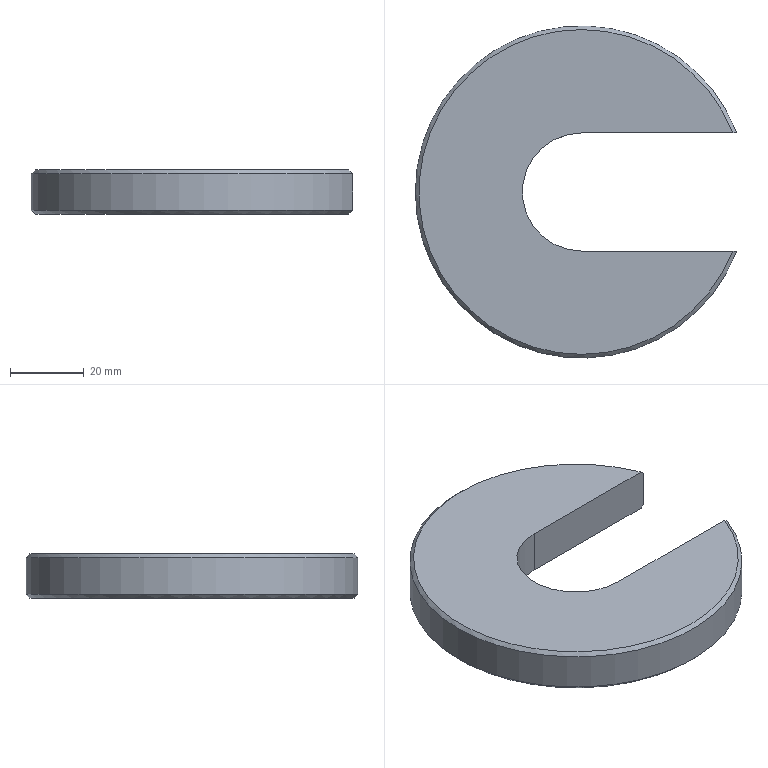Component | NX | QUICK_CHANGE_WASHER | 1 solid | 8 faces | box 87.06 x 90 x 12 mm | volume 54359 mm3 | plane 4 | cylinder 2 | cone 2 | commonest cylinder face diameters 32 x1 90 x1
STEP:
#1=CARTESIAN_POINT('',(0.,0.,0.));
#2=DIRECTION('',(0.,0.,1.));
#3=DIRECTION('',(1.,0.,0.));
#4=AXIS2_PLACEMENT_3D('',#1,#2,#3);
#5=CARTESIAN_POINT('',(42.059,-16.,129.));
#6=VERTEX_POINT('',#5);
#7=CARTESIAN_POINT('',(42.059,-16.,119.));
#8=VERTEX_POINT('',#7);
#9=CARTESIAN_POINT('',(42.059,-16.,130.));
#10=DIRECTION('',(0.,0.,-1.));
#11=VECTOR('',#10,1.);
#12=LINE('',#9,#11);
#13=CARTESIAN_POINT('',(42.059,-16.,130.));
#14=DIRECTION('',(0.,-1.,0.));
#15=DIRECTION('',(1.,0.,0.));
#16=AXIS2_PLACEMENT_3D('',#13,#14,#15);
#17=PLANE('',#16);
#18=CARTESIAN_POINT('',(0.,0.));
#19=DIRECTION('',(0.,-1.));
#20=VECTOR('',#19,1.);
#21=LINE('',#18,#20);
#22=(GEOMETRIC_REPRESENTATION_CONTEXT(2)PARAMETRIC_REPRESENTATION_CONTEXT()REPRESENTATION_CONTEXT('',''));
#23=DEFINITIONAL_REPRESENTATION('',(#21),#22);
#24=PCURVE('',#17,#23);
#25=CARTESIAN_POINT('',(-0.,0.,130.));
#26=DIRECTION('',(0.,0.,-1.));
#27=DIRECTION('',(0.,-1.,0.));
#28=AXIS2_PLACEMENT_3D('',#25,#26,#27);
#29=CYLINDRICAL_SURFACE('',#28,45.);
#30=CARTESIAN_POINT('',(-1.207,0.));
#31=DIRECTION('',(0.,1.));
#32=VECTOR('',#31,1.);
#33=LINE('',#30,#32);
#34=(GEOMETRIC_REPRESENTATION_CONTEXT(2)PARAMETRIC_REPRESENTATION_CONTEXT()REPRESENTATION_CONTEXT('',''));
#35=DEFINITIONAL_REPRESENTATION('',(#33),#34);
#36=PCURVE('',#29,#35);
#37=SURFACE_CURVE('',#12,(#24,#36),.PCURVE_S1.);
#38=EDGE_CURVE('',#6,#8,#37,.T.);
#39=ORIENTED_EDGE('',*,*,#38,.T.);
#40=CARTESIAN_POINT('',(40.988,-16.,118.));
#41=VERTEX_POINT('',#40);
#42=CARTESIAN_POINT('',(42.059,-16.,119.));
#43=CARTESIAN_POINT('',(41.703,-16.,118.666));
#44=CARTESIAN_POINT('',(41.345,-16.,118.333));
#45=CARTESIAN_POINT('',(40.988,-16.,118.));
#46=B_SPLINE_CURVE_WITH_KNOTS('',3,(#42,#43,#44,#45),.UNSPECIFIED.,.F.,.F.,(4,4),(0.,1.),.PIECEWISE_BEZIER_KNOTS.);
#47=CARTESIAN_POINT('',(0.,-11.));
#48=CARTESIAN_POINT('',(-0.357,-11.334));
#49=CARTESIAN_POINT('',(-0.7142,-11.667));
#50=CARTESIAN_POINT('',(-1.072,-12.));
#51=B_SPLINE_CURVE_WITH_KNOTS('',3,(#47,#48,#49,#50),.UNSPECIFIED.,.F.,.F.,(4,4),(0.,1.),.PIECEWISE_BEZIER_KNOTS.);
#52=(GEOMETRIC_REPRESENTATION_CONTEXT(2)PARAMETRIC_REPRESENTATION_CONTEXT()REPRESENTATION_CONTEXT('',''));
#53=DEFINITIONAL_REPRESENTATION('',(#51),#52);
#54=PCURVE('',#17,#53);
#55=CARTESIAN_POINT('',(-0.,0.,119.));
#56=DIRECTION('',(0.,0.,1.));
#57=DIRECTION('',(0.,1.,0.));
#58=AXIS2_PLACEMENT_3D('',#55,#56,#57);
#59=CONICAL_SURFACE('',#58,45.,0.7854);
#60=CARTESIAN_POINT('',(4.349,0.));
#61=CARTESIAN_POINT('',(4.34,-1.));
#62=B_SPLINE_CURVE_WITH_KNOTS('',1,(#60,#61),.UNSPECIFIED.,.F.,.F.,(2,2),(0.,1.),.PIECEWISE_BEZIER_KNOTS.);
#63=(GEOMETRIC_REPRESENTATION_CONTEXT(2)PARAMETRIC_REPRESENTATION_CONTEXT()REPRESENTATION_CONTEXT('',''));
#64=DEFINITIONAL_REPRESENTATION('',(#62),#63);
#65=PCURVE('',#59,#64);
#66=SURFACE_CURVE('',#46,(#54,#65),.PCURVE_S1.);
#67=EDGE_CURVE('',#8,#41,#66,.T.);
#68=ORIENTED_EDGE('',*,*,#67,.T.);
#69=CARTESIAN_POINT('',(-0.,-16.,118.));
#70=VERTEX_POINT('',#69);
#71=CARTESIAN_POINT('',(42.059,-16.,118.));
#72=DIRECTION('',(-1.,-0.,0.));
#73=VECTOR('',#72,1.);
#74=LINE('',#71,#73);
#75=CARTESIAN_POINT('',(0.,-12.));
#76=DIRECTION('',(-1.,0.));
#77=VECTOR('',#76,1.);
#78=LINE('',#75,#77);
#79=(GEOMETRIC_REPRESENTATION_CONTEXT(2)PARAMETRIC_REPRESENTATION_CONTEXT()REPRESENTATION_CONTEXT('',''));
#80=DEFINITIONAL_REPRESENTATION('',(#78),#79);
#81=PCURVE('',#17,#80);
#82=CARTESIAN_POINT('',(-0.,0.,118.));
#83=DIRECTION('',(0.,0.,-1.));
#84=DIRECTION('',(0.,-1.,0.));
#85=AXIS2_PLACEMENT_3D('',#82,#83,#84);
#86=PLANE('',#85);
#87=CARTESIAN_POINT('',(16.,-42.059));
#88=DIRECTION('',(0.,1.));
#89=VECTOR('',#88,1.);
#90=LINE('',#87,#89);
#91=(GEOMETRIC_REPRESENTATION_CONTEXT(2)PARAMETRIC_REPRESENTATION_CONTEXT()REPRESENTATION_CONTEXT('',''));
#92=DEFINITIONAL_REPRESENTATION('',(#90),#91);
#93=PCURVE('',#86,#92);
#94=SURFACE_CURVE('',#74,(#81,#93),.PCURVE_S1.);
#95=EDGE_CURVE('',#41,#70,#94,.T.);
#96=ORIENTED_EDGE('',*,*,#95,.T.);
#97=CARTESIAN_POINT('',(-0.,-16.,130.));
#98=VERTEX_POINT('',#97);
#99=CARTESIAN_POINT('',(-0.,-16.,130.));
#100=DIRECTION('',(0.,0.,-1.));
#101=VECTOR('',#100,1.);
#102=LINE('',#99,#101);
#103=CARTESIAN_POINT('',(-42.059,0.));
#104=DIRECTION('',(0.,-1.));
#105=VECTOR('',#104,1.);
#106=LINE('',#103,#105);
#107=(GEOMETRIC_REPRESENTATION_CONTEXT(2)PARAMETRIC_REPRESENTATION_CONTEXT()REPRESENTATION_CONTEXT('',''));
#108=DEFINITIONAL_REPRESENTATION('',(#106),#107);
#109=PCURVE('',#17,#108);
#110=CARTESIAN_POINT('',(-0.,0.,130.));
#111=DIRECTION('',(0.,0.,-1.));
#112=DIRECTION('',(0.,-1.,0.));
#113=AXIS2_PLACEMENT_3D('',#110,#111,#112);
#114=CYLINDRICAL_SURFACE('',#113,16.);
#115=CARTESIAN_POINT('',(0.,0.));
#116=DIRECTION('',(0.,1.));
#117=VECTOR('',#116,1.);
#118=LINE('',#115,#117);
#119=(GEOMETRIC_REPRESENTATION_CONTEXT(2)PARAMETRIC_REPRESENTATION_CONTEXT()REPRESENTATION_CONTEXT('',''));
#120=DEFINITIONAL_REPRESENTATION('',(#118),#119);
#121=PCURVE('',#114,#120);
#122=SURFACE_CURVE('',#102,(#109,#121),.PCURVE_S1.);
#123=EDGE_CURVE('',#98,#70,#122,.T.);
#124=ORIENTED_EDGE('',*,*,#123,.F.);
#125=CARTESIAN_POINT('',(40.988,-16.,130.));
#126=VERTEX_POINT('',#125);
#127=CARTESIAN_POINT('',(42.059,-16.,130.));
#128=DIRECTION('',(-1.,-0.,0.));
#129=VECTOR('',#128,1.);
#130=LINE('',#127,#129);
#131=CARTESIAN_POINT('',(0.,0.));
#132=DIRECTION('',(-1.,0.));
#133=VECTOR('',#132,1.);
#134=LINE('',#131,#133);
#135=(GEOMETRIC_REPRESENTATION_CONTEXT(2)PARAMETRIC_REPRESENTATION_CONTEXT()REPRESENTATION_CONTEXT('',''));
#136=DEFINITIONAL_REPRESENTATION('',(#134),#135);
#137=PCURVE('',#17,#136);
#138=CARTESIAN_POINT('',(-0.,0.,130.));
#139=DIRECTION('',(0.,0.,-1.));
#140=DIRECTION('',(0.,-1.,0.));
#141=AXIS2_PLACEMENT_3D('',#138,#139,#140);
#142=PLANE('',#141);
#143=CARTESIAN_POINT('',(16.,-42.059));
#144=DIRECTION('',(0.,1.));
#145=VECTOR('',#144,1.);
#146=LINE('',#143,#145);
#147=(GEOMETRIC_REPRESENTATION_CONTEXT(2)PARAMETRIC_REPRESENTATION_CONTEXT()REPRESENTATION_CONTEXT('',''));
#148=DEFINITIONAL_REPRESENTATION('',(#146),#147);
#149=PCURVE('',#142,#148);
#150=SURFACE_CURVE('',#130,(#137,#149),.PCURVE_S1.);
#151=EDGE_CURVE('',#126,#98,#150,.T.);
#152=ORIENTED_EDGE('',*,*,#151,.F.);
#153=CARTESIAN_POINT('',(40.988,-16.,130.));
#154=CARTESIAN_POINT('',(41.345,-16.,129.667));
#155=CARTESIAN_POINT('',(41.703,-16.,129.334));
#156=CARTESIAN_POINT('',(42.059,-16.,129.));
#157=B_SPLINE_CURVE_WITH_KNOTS('',3,(#153,#154,#155,#156),.UNSPECIFIED.,.F.,.F.,(4,4),(0.,1.),.PIECEWISE_BEZIER_KNOTS.);
#158=CARTESIAN_POINT('',(-1.072,0.));
#159=CARTESIAN_POINT('',(-0.7142,-0.333));
#160=CARTESIAN_POINT('',(-0.357,-0.6664));
#161=CARTESIAN_POINT('',(0.,-1.));
#162=B_SPLINE_CURVE_WITH_KNOTS('',3,(#158,#159,#160,#161),.UNSPECIFIED.,.F.,.F.,(4,4),(0.,1.),.PIECEWISE_BEZIER_KNOTS.);
#163=(GEOMETRIC_REPRESENTATION_CONTEXT(2)PARAMETRIC_REPRESENTATION_CONTEXT()REPRESENTATION_CONTEXT('',''));
#164=DEFINITIONAL_REPRESENTATION('',(#162),#163);
#165=PCURVE('',#17,#164);
#166=CARTESIAN_POINT('',(-0.,0.,130.));
#167=DIRECTION('',(0.,0.,-1.));
#168=DIRECTION('',(0.,-1.,0.));
#169=AXIS2_PLACEMENT_3D('',#166,#167,#168);
#170=CONICAL_SURFACE('',#169,44.,0.7854);
#171=CARTESIAN_POINT('',(-1.199,0.));
#172=CARTESIAN_POINT('',(-1.207,1.));
#173=B_SPLINE_CURVE_WITH_KNOTS('',1,(#171,#172),.UNSPECIFIED.,.F.,.F.,(2,2),(0.,1.),.PIECEWISE_BEZIER_KNOTS.);
#174=(GEOMETRIC_REPRESENTATION_CONTEXT(2)PARAMETRIC_REPRESENTATION_CONTEXT()REPRESENTATION_CONTEXT('',''));
#175=DEFINITIONAL_REPRESENTATION('',(#173),#174);
#176=PCURVE('',#170,#175);
#177=SURFACE_CURVE('',#157,(#165,#176),.PCURVE_S1.);
#178=EDGE_CURVE('',#126,#6,#177,.T.);
#179=ORIENTED_EDGE('',*,*,#178,.T.);
#180=EDGE_LOOP('',(#39,#68,#96,#124,#152,#179));
#181=FACE_BOUND('',#180,.T.);
#182=ADVANCED_FACE('',(#181),#17,.F.);
#183=ORIENTED_EDGE('',*,*,#123,.F.);
#184=CARTESIAN_POINT('',(-0.,16.,130.));
#185=VERTEX_POINT('',#184);
#186=CARTESIAN_POINT('',(-0.,0.,130.));
#187=DIRECTION('',(0.,0.,-1.));
#188=DIRECTION('',(-0.,1.,0.));
#189=AXIS2_PLACEMENT_3D('',#186,#187,#188);
#190=CIRCLE('',#189,16.);
#191=CARTESIAN_POINT('',(-3.142,0.));
#192=DIRECTION('',(1.,0.));
#193=VECTOR('',#192,1.);
#194=LINE('',#191,#193);
#195=(GEOMETRIC_REPRESENTATION_CONTEXT(2)PARAMETRIC_REPRESENTATION_CONTEXT()REPRESENTATION_CONTEXT('',''));
#196=DEFINITIONAL_REPRESENTATION('',(#194),#195);
#197=PCURVE('',#114,#196);
#198=CARTESIAN_POINT('',(0.,0.));
#199=DIRECTION('',(-1.,0.));
#200=AXIS2_PLACEMENT_2D('',#198,#199);
#201=CIRCLE('',#200,16.);
#202=(GEOMETRIC_REPRESENTATION_CONTEXT(2)PARAMETRIC_REPRESENTATION_CONTEXT()REPRESENTATION_CONTEXT('',''));
#203=DEFINITIONAL_REPRESENTATION('',(#201),#202);
#204=PCURVE('',#142,#203);
#205=SURFACE_CURVE('',#190,(#197,#204),.PCURVE_S1.);
#206=EDGE_CURVE('',#98,#185,#205,.T.);
#207=ORIENTED_EDGE('',*,*,#206,.T.);
#208=CARTESIAN_POINT('',(-0.,16.,118.));
#209=VERTEX_POINT('',#208);
#210=CARTESIAN_POINT('',(-0.,16.,130.));
#211=DIRECTION('',(0.,0.,-1.));
#212=VECTOR('',#211,1.);
#213=LINE('',#210,#212);
#214=CARTESIAN_POINT('',(3.142,0.));
#215=DIRECTION('',(0.,1.));
#216=VECTOR('',#215,1.);
#217=LINE('',#214,#216);
#218=(GEOMETRIC_REPRESENTATION_CONTEXT(2)PARAMETRIC_REPRESENTATION_CONTEXT()REPRESENTATION_CONTEXT('',''));
#219=DEFINITIONAL_REPRESENTATION('',(#217),#218);
#220=PCURVE('',#114,#219);
#221=CARTESIAN_POINT('',(-0.,16.,130.));
#222=DIRECTION('',(-0.,1.,0.));
#223=DIRECTION('',(-1.,-0.,0.));
#224=AXIS2_PLACEMENT_3D('',#221,#222,#223);
#225=PLANE('',#224);
#226=CARTESIAN_POINT('',(0.,0.));
#227=DIRECTION('',(0.,-1.));
#228=VECTOR('',#227,1.);
#229=LINE('',#226,#228);
#230=(GEOMETRIC_REPRESENTATION_CONTEXT(2)PARAMETRIC_REPRESENTATION_CONTEXT()REPRESENTATION_CONTEXT('',''));
#231=DEFINITIONAL_REPRESENTATION('',(#229),#230);
#232=PCURVE('',#225,#231);
#233=SURFACE_CURVE('',#213,(#220,#232),.PCURVE_S1.);
#234=EDGE_CURVE('',#185,#209,#233,.T.);
#235=ORIENTED_EDGE('',*,*,#234,.T.);
#236=CARTESIAN_POINT('',(-0.,0.,118.));
#237=DIRECTION('',(0.,0.,-1.));
#238=DIRECTION('',(-0.,1.,0.));
#239=AXIS2_PLACEMENT_3D('',#236,#237,#238);
#240=CIRCLE('',#239,16.);
#241=CARTESIAN_POINT('',(-3.142,12.));
#242=DIRECTION('',(1.,0.));
#243=VECTOR('',#242,1.);
#244=LINE('',#241,#243);
#245=(GEOMETRIC_REPRESENTATION_CONTEXT(2)PARAMETRIC_REPRESENTATION_CONTEXT()REPRESENTATION_CONTEXT('',''));
#246=DEFINITIONAL_REPRESENTATION('',(#244),#245);
#247=PCURVE('',#114,#246);
#248=CARTESIAN_POINT('',(0.,0.));
#249=DIRECTION('',(-1.,0.));
#250=AXIS2_PLACEMENT_2D('',#248,#249);
#251=CIRCLE('',#250,16.);
#252=(GEOMETRIC_REPRESENTATION_CONTEXT(2)PARAMETRIC_REPRESENTATION_CONTEXT()REPRESENTATION_CONTEXT('',''));
#253=DEFINITIONAL_REPRESENTATION('',(#251),#252);
#254=PCURVE('',#86,#253);
#255=SURFACE_CURVE('',#240,(#247,#254),.PCURVE_S1.);
#256=EDGE_CURVE('',#70,#209,#255,.T.);
#257=ORIENTED_EDGE('',*,*,#256,.F.);
#258=EDGE_LOOP('',(#183,#207,#235,#257));
#259=FACE_BOUND('',#258,.F.);
#260=ADVANCED_FACE('',(#259),#114,.F.);
#261=CARTESIAN_POINT('',(40.988,16.,118.));
#262=VERTEX_POINT('',#261);
#263=CARTESIAN_POINT('',(-0.,16.,118.));
#264=DIRECTION('',(1.,0.,0.));
#265=VECTOR('',#264,1.);
#266=LINE('',#263,#265);
#267=CARTESIAN_POINT('',(0.,-12.));
#268=DIRECTION('',(-1.,0.));
#269=VECTOR('',#268,1.);
#270=LINE('',#267,#269);
#271=(GEOMETRIC_REPRESENTATION_CONTEXT(2)PARAMETRIC_REPRESENTATION_CONTEXT()REPRESENTATION_CONTEXT('',''));
#272=DEFINITIONAL_REPRESENTATION('',(#270),#271);
#273=PCURVE('',#225,#272);
#274=CARTESIAN_POINT('',(-16.,-0.));
#275=DIRECTION('',(-0.,-1.));
#276=VECTOR('',#275,1.);
#277=LINE('',#274,#276);
#278=(GEOMETRIC_REPRESENTATION_CONTEXT(2)PARAMETRIC_REPRESENTATION_CONTEXT()REPRESENTATION_CONTEXT('',''));
#279=DEFINITIONAL_REPRESENTATION('',(#277),#278);
#280=PCURVE('',#86,#279);
#281=SURFACE_CURVE('',#266,(#273,#280),.PCURVE_S1.);
#282=EDGE_CURVE('',#209,#262,#281,.T.);
#283=ORIENTED_EDGE('',*,*,#282,.T.);
#284=CARTESIAN_POINT('',(42.059,16.,119.));
#285=VERTEX_POINT('',#284);
#286=CARTESIAN_POINT('',(40.988,16.,118.));
#287=CARTESIAN_POINT('',(41.345,16.,118.333));
#288=CARTESIAN_POINT('',(41.703,16.,118.666));
#289=CARTESIAN_POINT('',(42.059,16.,119.));
#290=B_SPLINE_CURVE_WITH_KNOTS('',3,(#286,#287,#288,#289),.UNSPECIFIED.,.F.,.F.,(4,4),(0.,1.),.PIECEWISE_BEZIER_KNOTS.);
#291=CARTESIAN_POINT('',(-40.988,-12.));
#292=CARTESIAN_POINT('',(-41.345,-11.667));
#293=CARTESIAN_POINT('',(-41.703,-11.334));
#294=CARTESIAN_POINT('',(-42.059,-11.));
#295=B_SPLINE_CURVE_WITH_KNOTS('',3,(#291,#292,#293,#294),.UNSPECIFIED.,.F.,.F.,(4,4),(0.,1.),.PIECEWISE_BEZIER_KNOTS.);
#296=(GEOMETRIC_REPRESENTATION_CONTEXT(2)PARAMETRIC_REPRESENTATION_CONTEXT()REPRESENTATION_CONTEXT('',''));
#297=DEFINITIONAL_REPRESENTATION('',(#295),#296);
#298=PCURVE('',#225,#297);
#299=CARTESIAN_POINT('',(-1.199,-1.));
#300=CARTESIAN_POINT('',(-1.207,0.));
#301=B_SPLINE_CURVE_WITH_KNOTS('',1,(#299,#300),.UNSPECIFIED.,.F.,.F.,(2,2),(0.,1.),.PIECEWISE_BEZIER_KNOTS.);
#302=(GEOMETRIC_REPRESENTATION_CONTEXT(2)PARAMETRIC_REPRESENTATION_CONTEXT()REPRESENTATION_CONTEXT('',''));
#303=DEFINITIONAL_REPRESENTATION('',(#301),#302);
#304=PCURVE('',#59,#303);
#305=SURFACE_CURVE('',#290,(#298,#304),.PCURVE_S1.);
#306=EDGE_CURVE('',#262,#285,#305,.T.);
#307=ORIENTED_EDGE('',*,*,#306,.T.);
#308=CARTESIAN_POINT('',(42.059,16.,129.));
#309=VERTEX_POINT('',#308);
#310=CARTESIAN_POINT('',(42.059,16.,130.));
#311=DIRECTION('',(0.,0.,-1.));
#312=VECTOR('',#311,1.);
#313=LINE('',#310,#312);
#314=CARTESIAN_POINT('',(-42.059,0.));
#315=DIRECTION('',(0.,-1.));
#316=VECTOR('',#315,1.);
#317=LINE('',#314,#316);
#318=(GEOMETRIC_REPRESENTATION_CONTEXT(2)PARAMETRIC_REPRESENTATION_CONTEXT()REPRESENTATION_CONTEXT('',''));
#319=DEFINITIONAL_REPRESENTATION('',(#317),#318);
#320=PCURVE('',#225,#319);
#321=CARTESIAN_POINT('',(4.349,0.));
#322=DIRECTION('',(0.,1.));
#323=VECTOR('',#322,1.);
#324=LINE('',#321,#323);
#325=(GEOMETRIC_REPRESENTATION_CONTEXT(2)PARAMETRIC_REPRESENTATION_CONTEXT()REPRESENTATION_CONTEXT('',''));
#326=DEFINITIONAL_REPRESENTATION('',(#324),#325);
#327=PCURVE('',#29,#326);
#328=SURFACE_CURVE('',#313,(#320,#327),.PCURVE_S1.);
#329=EDGE_CURVE('',#309,#285,#328,.T.);
#330=ORIENTED_EDGE('',*,*,#329,.F.);
#331=CARTESIAN_POINT('',(40.988,16.,130.));
#332=VERTEX_POINT('',#331);
#333=CARTESIAN_POINT('',(42.059,16.,129.));
#334=CARTESIAN_POINT('',(41.703,16.,129.334));
#335=CARTESIAN_POINT('',(41.345,16.,129.667));
#336=CARTESIAN_POINT('',(40.988,16.,130.));
#337=B_SPLINE_CURVE_WITH_KNOTS('',3,(#333,#334,#335,#336),.UNSPECIFIED.,.F.,.F.,(4,4),(0.,1.),.PIECEWISE_BEZIER_KNOTS.);
#338=CARTESIAN_POINT('',(-42.059,-1.));
#339=CARTESIAN_POINT('',(-41.703,-0.6664));
#340=CARTESIAN_POINT('',(-41.345,-0.333));
#341=CARTESIAN_POINT('',(-40.988,0.));
#342=B_SPLINE_CURVE_WITH_KNOTS('',3,(#338,#339,#340,#341),.UNSPECIFIED.,.F.,.F.,(4,4),(0.,1.),.PIECEWISE_BEZIER_KNOTS.);
#343=(GEOMETRIC_REPRESENTATION_CONTEXT(2)PARAMETRIC_REPRESENTATION_CONTEXT()REPRESENTATION_CONTEXT('',''));
#344=DEFINITIONAL_REPRESENTATION('',(#342),#343);
#345=PCURVE('',#225,#344);
#346=CARTESIAN_POINT('',(4.349,1.));
#347=CARTESIAN_POINT('',(4.34,0.));
#348=B_SPLINE_CURVE_WITH_KNOTS('',1,(#346,#347),.UNSPECIFIED.,.F.,.F.,(2,2),(0.,1.),.PIECEWISE_BEZIER_KNOTS.);
#349=(GEOMETRIC_REPRESENTATION_CONTEXT(2)PARAMETRIC_REPRESENTATION_CONTEXT()REPRESENTATION_CONTEXT('',''));
#350=DEFINITIONAL_REPRESENTATION('',(#348),#349);
#351=PCURVE('',#170,#350);
#352=SURFACE_CURVE('',#337,(#345,#351),.PCURVE_S1.);
#353=EDGE_CURVE('',#309,#332,#352,.T.);
#354=ORIENTED_EDGE('',*,*,#353,.T.);
#355=CARTESIAN_POINT('',(-0.,16.,130.));
#356=DIRECTION('',(1.,0.,0.));
#357=VECTOR('',#356,1.);
#358=LINE('',#355,#357);
#359=CARTESIAN_POINT('',(0.,0.));
#360=DIRECTION('',(-1.,0.));
#361=VECTOR('',#360,1.);
#362=LINE('',#359,#361);
#363=(GEOMETRIC_REPRESENTATION_CONTEXT(2)PARAMETRIC_REPRESENTATION_CONTEXT()REPRESENTATION_CONTEXT('',''));
#364=DEFINITIONAL_REPRESENTATION('',(#362),#363);
#365=PCURVE('',#225,#364);
#366=CARTESIAN_POINT('',(-16.,-0.));
#367=DIRECTION('',(-0.,-1.));
#368=VECTOR('',#367,1.);
#369=LINE('',#366,#368);
#370=(GEOMETRIC_REPRESENTATION_CONTEXT(2)PARAMETRIC_REPRESENTATION_CONTEXT()REPRESENTATION_CONTEXT('',''));
#371=DEFINITIONAL_REPRESENTATION('',(#369),#370);
#372=PCURVE('',#142,#371);
#373=SURFACE_CURVE('',#358,(#365,#372),.PCURVE_S1.);
#374=EDGE_CURVE('',#185,#332,#373,.T.);
#375=ORIENTED_EDGE('',*,*,#374,.F.);
#376=ORIENTED_EDGE('',*,*,#234,.T.);
#377=EDGE_LOOP('',(#283,#307,#330,#354,#375,#376));
#378=FACE_BOUND('',#377,.T.);
#379=ADVANCED_FACE('',(#378),#225,.F.);
#380=ORIENTED_EDGE('',*,*,#329,.T.);
#381=CARTESIAN_POINT('',(-0.,0.,119.));
#382=DIRECTION('',(0.,0.,1.));
#383=DIRECTION('',(0.,-1.,0.));
#384=AXIS2_PLACEMENT_3D('',#381,#382,#383);
#385=CIRCLE('',#384,45.);
#386=CARTESIAN_POINT('',(6.283,11.));
#387=DIRECTION('',(-1.,0.));
#388=VECTOR('',#387,1.);
#389=LINE('',#386,#388);
#390=(GEOMETRIC_REPRESENTATION_CONTEXT(2)PARAMETRIC_REPRESENTATION_CONTEXT()REPRESENTATION_CONTEXT('',''));
#391=DEFINITIONAL_REPRESENTATION('',(#389),#390);
#392=PCURVE('',#29,#391);
#393=CARTESIAN_POINT('',(-3.142,-0.));
#394=DIRECTION('',(1.,0.));
#395=VECTOR('',#394,1.);
#396=LINE('',#393,#395);
#397=(GEOMETRIC_REPRESENTATION_CONTEXT(2)PARAMETRIC_REPRESENTATION_CONTEXT()REPRESENTATION_CONTEXT('',''));
#398=DEFINITIONAL_REPRESENTATION('',(#396),#397);
#399=PCURVE('',#59,#398);
#400=SURFACE_CURVE('',#385,(#392,#399),.PCURVE_S1.);
#401=EDGE_CURVE('',#285,#8,#400,.T.);
#402=ORIENTED_EDGE('',*,*,#401,.T.);
#403=ORIENTED_EDGE('',*,*,#38,.F.);
#404=CARTESIAN_POINT('',(-0.,0.,129.));
#405=DIRECTION('',(0.,0.,-1.));
#406=DIRECTION('',(0.,-1.,0.));
#407=AXIS2_PLACEMENT_3D('',#404,#405,#406);
#408=CIRCLE('',#407,45.);
#409=CARTESIAN_POINT('',(-6.283,1.));
#410=DIRECTION('',(1.,0.));
#411=VECTOR('',#410,1.);
#412=LINE('',#409,#411);
#413=(GEOMETRIC_REPRESENTATION_CONTEXT(2)PARAMETRIC_REPRESENTATION_CONTEXT()REPRESENTATION_CONTEXT('',''));
#414=DEFINITIONAL_REPRESENTATION('',(#412),#413);
#415=PCURVE('',#29,#414);
#416=CARTESIAN_POINT('',(-6.283,1.));
#417=DIRECTION('',(1.,0.));
#418=VECTOR('',#417,1.);
#419=LINE('',#416,#418);
#420=(GEOMETRIC_REPRESENTATION_CONTEXT(2)PARAMETRIC_REPRESENTATION_CONTEXT()REPRESENTATION_CONTEXT('',''));
#421=DEFINITIONAL_REPRESENTATION('',(#419),#420);
#422=PCURVE('',#170,#421);
#423=SURFACE_CURVE('',#408,(#415,#422),.PCURVE_S1.);
#424=EDGE_CURVE('',#6,#309,#423,.T.);
#425=ORIENTED_EDGE('',*,*,#424,.T.);
#426=EDGE_LOOP('',(#380,#402,#403,#425));
#427=FACE_BOUND('',#426,.T.);
#428=ADVANCED_FACE('',(#427),#29,.T.);
#429=ORIENTED_EDGE('',*,*,#374,.T.);
#430=CARTESIAN_POINT('',(-0.,0.,130.));
#431=DIRECTION('',(0.,0.,1.));
#432=DIRECTION('',(0.,-1.,0.));
#433=AXIS2_PLACEMENT_3D('',#430,#431,#432);
#434=CIRCLE('',#433,44.);
#435=CARTESIAN_POINT('',(44.,0.));
#436=CARTESIAN_POINT('',(44.,-76.21));
#437=CARTESIAN_POINT('',(-22.,-38.105));
#438=CARTESIAN_POINT('',(-88.,-0.));
#439=CARTESIAN_POINT('',(-22.,38.105));
#440=CARTESIAN_POINT('',(44.,76.21));
#441=CARTESIAN_POINT('',(44.,0.));
#442=(BOUNDED_CURVE()B_SPLINE_CURVE(2,(#435,#436,#437,#438,#439,#440,#441),.UNSPECIFIED.,.T.,.F.)B_SPLINE_CURVE_WITH_KNOTS((1,2,2,2,2,1),(-2.094,0.,2.094,4.189,6.283,8.378),.UNSPECIFIED.)CURVE()GEOMETRIC_REPRESENTATION_ITEM()RATIONAL_B_SPLINE_CURVE((1.,0.5,1.,0.5,1.,0.5,1.))REPRESENTATION_ITEM(''));
#443=(GEOMETRIC_REPRESENTATION_CONTEXT(2)PARAMETRIC_REPRESENTATION_CONTEXT()REPRESENTATION_CONTEXT('',''));
#444=DEFINITIONAL_REPRESENTATION('',(#442),#443);
#445=PCURVE('',#142,#444);
#446=CARTESIAN_POINT('',(6.283,-0.));
#447=DIRECTION('',(-1.,0.));
#448=VECTOR('',#447,1.);
#449=LINE('',#446,#448);
#450=(GEOMETRIC_REPRESENTATION_CONTEXT(2)PARAMETRIC_REPRESENTATION_CONTEXT()REPRESENTATION_CONTEXT('',''));
#451=DEFINITIONAL_REPRESENTATION('',(#449),#450);
#452=PCURVE('',#170,#451);
#453=SURFACE_CURVE('',#434,(#445,#452),.PCURVE_S1.);
#454=EDGE_CURVE('',#332,#126,#453,.T.);
#455=ORIENTED_EDGE('',*,*,#454,.T.);
#456=ORIENTED_EDGE('',*,*,#151,.T.);
#457=ORIENTED_EDGE('',*,*,#206,.T.);
#458=EDGE_LOOP('',(#429,#455,#456,#457));
#459=FACE_BOUND('',#458,.T.);
#460=ADVANCED_FACE('',(#459),#142,.F.);
#461=ORIENTED_EDGE('',*,*,#95,.F.);
#462=CARTESIAN_POINT('',(-0.,0.,118.));
#463=DIRECTION('',(0.,0.,-1.));
#464=DIRECTION('',(0.,-1.,0.));
#465=AXIS2_PLACEMENT_3D('',#462,#463,#464);
#466=CIRCLE('',#465,44.);
#467=CARTESIAN_POINT('',(0.,0.));
#468=DIRECTION('',(1.,0.));
#469=AXIS2_PLACEMENT_2D('',#467,#468);
#470=CIRCLE('',#469,44.);
#471=(GEOMETRIC_REPRESENTATION_CONTEXT(2)PARAMETRIC_REPRESENTATION_CONTEXT()REPRESENTATION_CONTEXT('',''));
#472=DEFINITIONAL_REPRESENTATION('',(#470),#471);
#473=PCURVE('',#86,#472);
#474=CARTESIAN_POINT('',(9.425,-1.));
#475=DIRECTION('',(-1.,0.));
#476=VECTOR('',#475,1.);
#477=LINE('',#474,#476);
#478=(GEOMETRIC_REPRESENTATION_CONTEXT(2)PARAMETRIC_REPRESENTATION_CONTEXT()REPRESENTATION_CONTEXT('',''));
#479=DEFINITIONAL_REPRESENTATION('',(#477),#478);
#480=PCURVE('',#59,#479);
#481=SURFACE_CURVE('',#466,(#473,#480),.PCURVE_S1.);
#482=EDGE_CURVE('',#41,#262,#481,.T.);
#483=ORIENTED_EDGE('',*,*,#482,.T.);
#484=ORIENTED_EDGE('',*,*,#282,.F.);
#485=ORIENTED_EDGE('',*,*,#256,.F.);
#486=EDGE_LOOP('',(#461,#483,#484,#485));
#487=FACE_BOUND('',#486,.T.);
#488=ADVANCED_FACE('',(#487),#86,.T.);
#489=ORIENTED_EDGE('',*,*,#306,.F.);
#490=ORIENTED_EDGE('',*,*,#482,.F.);
#491=ORIENTED_EDGE('',*,*,#67,.F.);
#492=ORIENTED_EDGE('',*,*,#401,.F.);
#493=EDGE_LOOP('',(#489,#490,#491,#492));
#494=FACE_BOUND('',#493,.T.);
#495=ADVANCED_FACE('',(#494),#59,.T.);
#496=ORIENTED_EDGE('',*,*,#353,.F.);
#497=ORIENTED_EDGE('',*,*,#424,.F.);
#498=ORIENTED_EDGE('',*,*,#178,.F.);
#499=ORIENTED_EDGE('',*,*,#454,.F.);
#500=EDGE_LOOP('',(#496,#497,#498,#499));
#501=FACE_BOUND('',#500,.T.);
#502=ADVANCED_FACE('',(#501),#170,.T.);
#503=CLOSED_SHELL('',(#182,#260,#379,#428,#460,#488,#495,#502));
#504=MANIFOLD_SOLID_BREP('',#503);
#505=(LENGTH_UNIT()NAMED_UNIT(*)SI_UNIT(.MILLI.,.METRE.));
#506=UNCERTAINTY_MEASURE_WITH_UNIT(LENGTH_MEASURE(0.001),#505,'','');
#507=(NAMED_UNIT(*)PLANE_ANGLE_UNIT()SI_UNIT($,.RADIAN.));
#508=(NAMED_UNIT(*)SI_UNIT($,.STERADIAN.)SOLID_ANGLE_UNIT());
#509=(GEOMETRIC_REPRESENTATION_CONTEXT(3)GLOBAL_UNCERTAINTY_ASSIGNED_CONTEXT((#506))GLOBAL_UNIT_ASSIGNED_CONTEXT((#505,#507,#508))REPRESENTATION_CONTEXT('',''));
#510=ADVANCED_BREP_SHAPE_REPRESENTATION('',(#4,#504),#509);